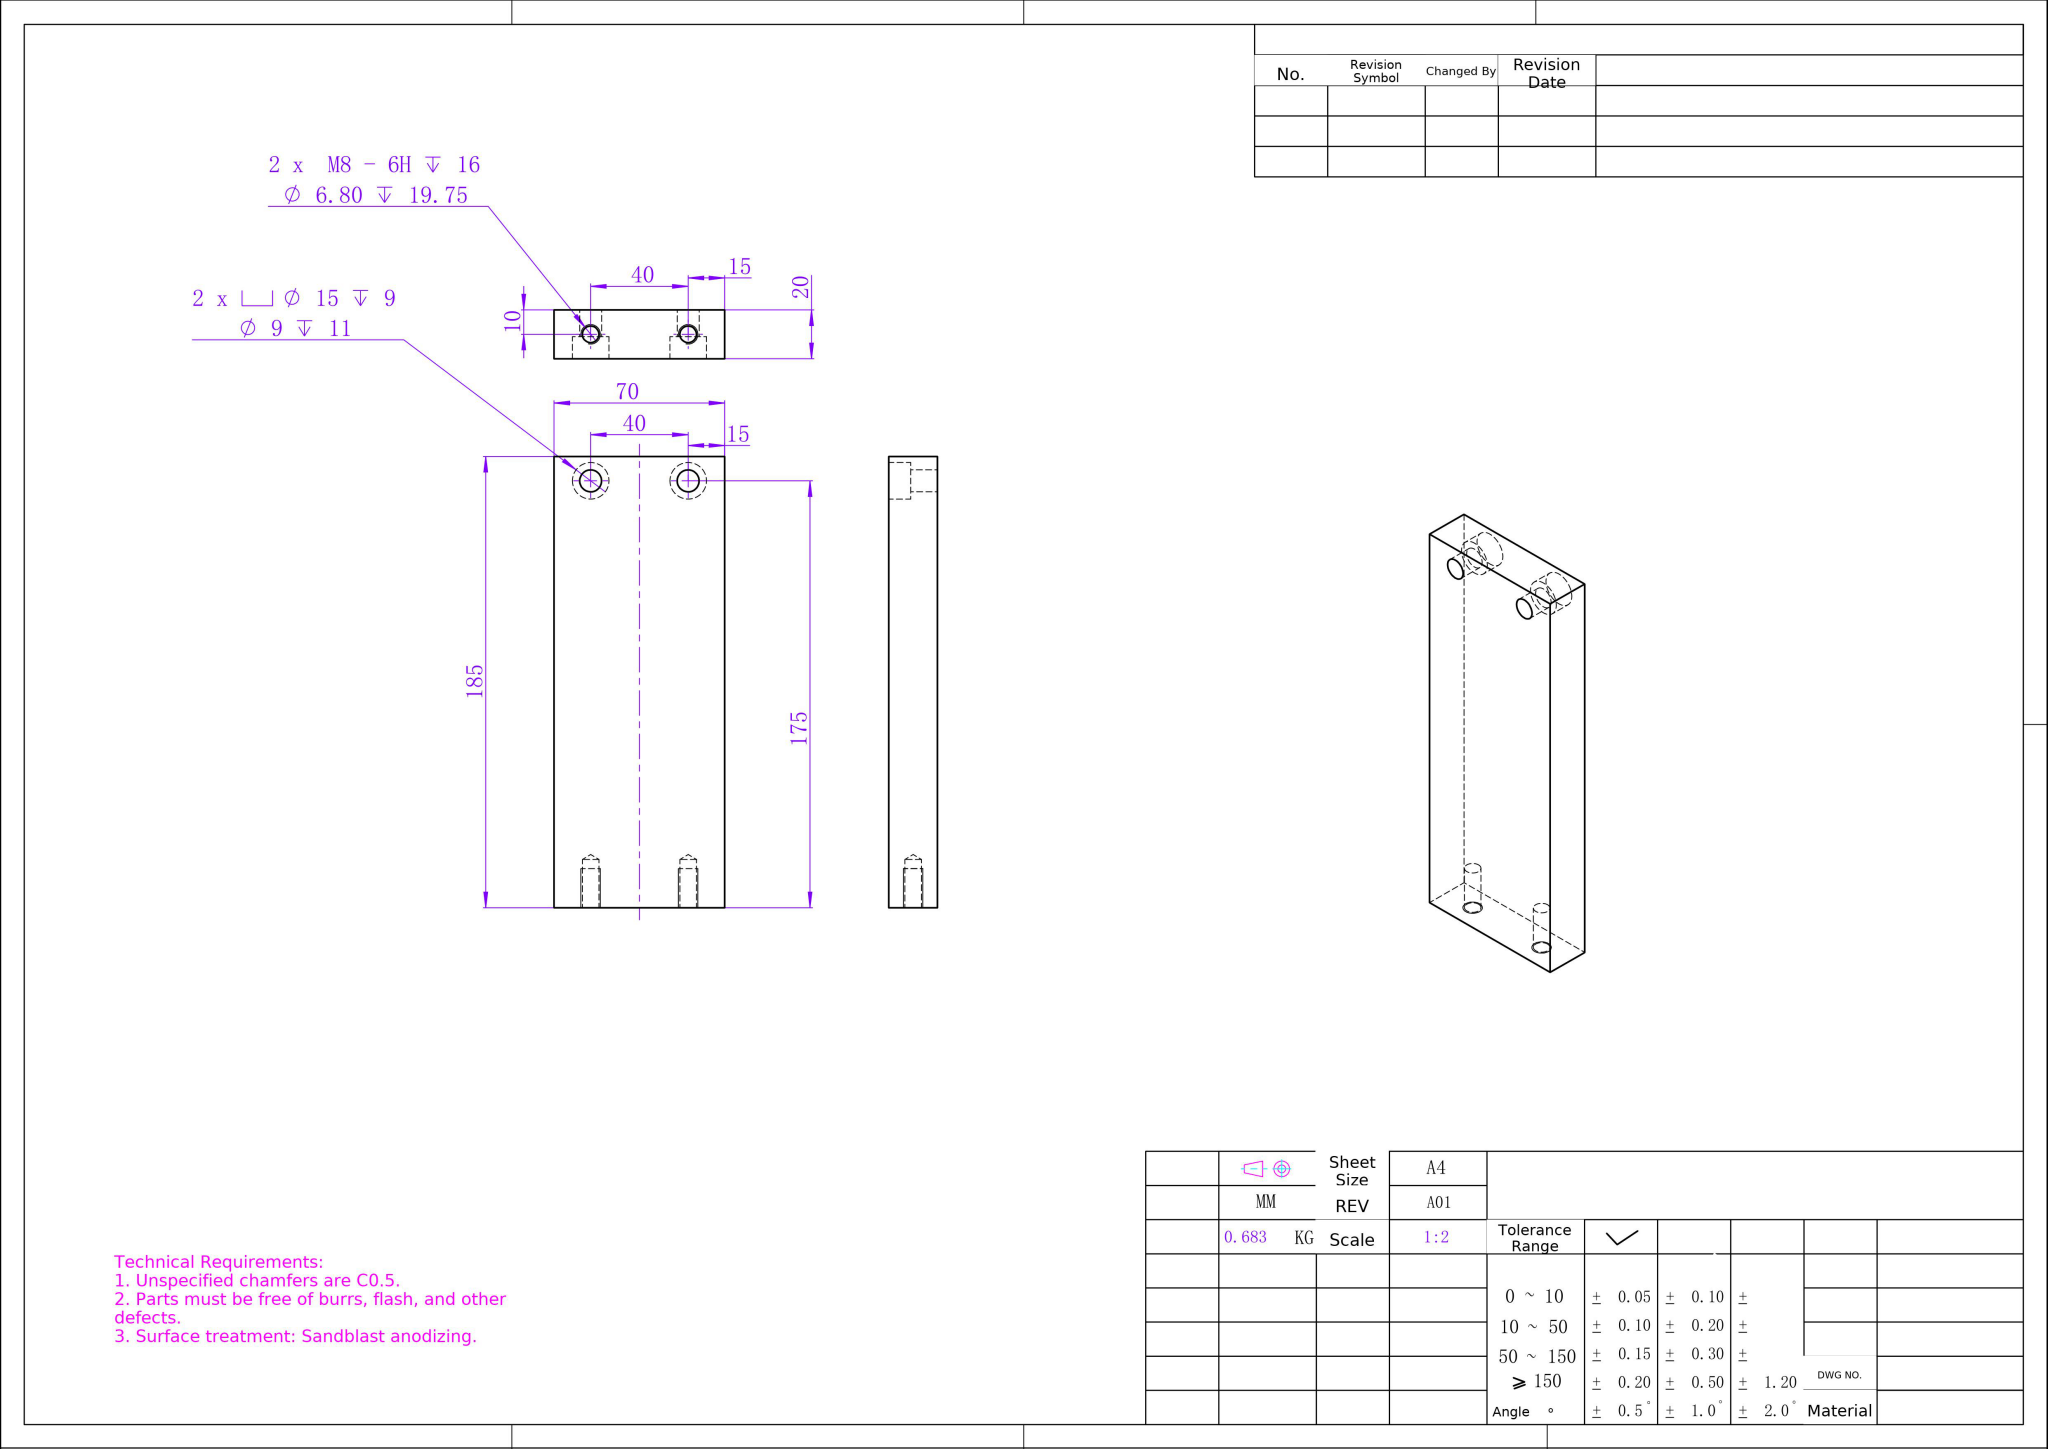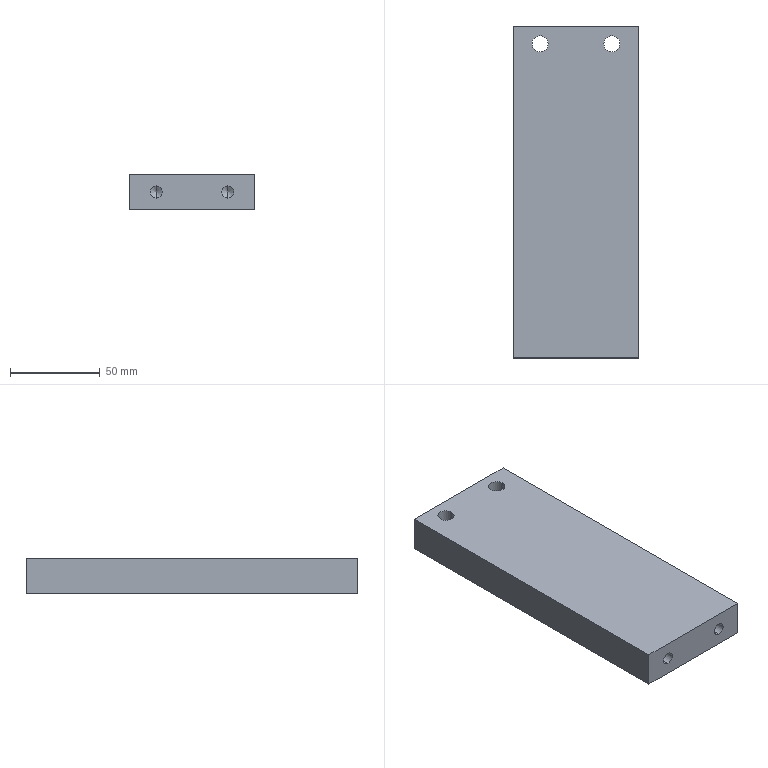Part | NX | mm | 1 solid | 24 faces | box 70 x 185 x 20 mm | volume 252936 mm3 | cylinder 12 | plane 8 | cone 4 | commonest cylinder face diameters 6.8 x4 9 x4 15 x4
STEP:
#1=COLOUR_RGB('',0.0902,1.,0.902);
#2=FILL_AREA_STYLE_COLOUR('',#1);
#3=FILL_AREA_STYLE('',(#2));
#4=SURFACE_STYLE_FILL_AREA(#3);
#5=SURFACE_SIDE_STYLE('',(#4));
#6=SURFACE_STYLE_USAGE(.BOTH.,#5);
#7=PRESENTATION_STYLE_ASSIGNMENT((#6));
#8=CARTESIAN_POINT('',(-695.,514.75,-6.6));
#9=VERTEX_POINT('',#8);
#10=CARTESIAN_POINT('',(-695.,514.75,-13.4));
#11=VERTEX_POINT('',#10);
#12=CARTESIAN_POINT('',(-695.,514.75,-10.));
#13=DIRECTION('',(0.,-1.,0.));
#14=DIRECTION('',(0.,0.,-1.));
#15=AXIS2_PLACEMENT_3D('',#12,#13,#14);
#16=CIRCLE('',#15,3.4);
#17=EDGE_CURVE('',#9,#11,#16,.T.);
#18=ORIENTED_EDGE('',*,*,#17,.F.);
#19=CARTESIAN_POINT('',(-695.,495.,-6.6));
#20=VERTEX_POINT('',#19);
#21=CARTESIAN_POINT('',(-695.,495.,-6.6));
#22=DIRECTION('',(0.,-1.,0.));
#23=VECTOR('',#22,1000.);
#24=LINE('',#21,#23);
#25=EDGE_CURVE('',#9,#20,#24,.T.);
#26=ORIENTED_EDGE('',*,*,#25,.T.);
#27=CARTESIAN_POINT('',(-695.,495.,-13.4));
#28=VERTEX_POINT('',#27);
#29=CARTESIAN_POINT('',(-695.,495.,-10.));
#30=DIRECTION('',(0.,-1.,0.));
#31=DIRECTION('',(0.,0.,-1.));
#32=AXIS2_PLACEMENT_3D('',#29,#30,#31);
#33=CIRCLE('',#32,3.4);
#34=EDGE_CURVE('',#20,#28,#33,.T.);
#35=ORIENTED_EDGE('',*,*,#34,.T.);
#36=CARTESIAN_POINT('',(-695.,495.,-13.4));
#37=DIRECTION('',(0.,-1.,0.));
#38=VECTOR('',#37,1000.);
#39=LINE('',#36,#38);
#40=EDGE_CURVE('',#11,#28,#39,.T.);
#41=ORIENTED_EDGE('',*,*,#40,.F.);
#42=EDGE_LOOP('',(#18,#26,#35,#41));
#43=FACE_OUTER_BOUND('',#42,.T.);
#44=CARTESIAN_POINT('',(-695.,495.,-10.));
#45=DIRECTION('',(0.,-1.,0.));
#46=DIRECTION('',(0.,0.,-1.));
#47=AXIS2_PLACEMENT_3D('',#44,#45,#46);
#48=CYLINDRICAL_SURFACE('',#47,3.4);
#49=ADVANCED_FACE('',(#43),#48,.F.);
#50=STYLED_ITEM('',(#7),#49);
#51=PRESENTATION_LAYER_ASSIGNMENT('','',(#50));
#52=COLOUR_RGB('',0.0902,1.,0.902);
#53=FILL_AREA_STYLE_COLOUR('',#52);
#54=FILL_AREA_STYLE('',(#53));
#55=SURFACE_STYLE_FILL_AREA(#54);
#56=SURFACE_SIDE_STYLE('',(#55));
#57=SURFACE_STYLE_USAGE(.BOTH.,#56);
#58=PRESENTATION_STYLE_ASSIGNMENT((#57));
#59=ORIENTED_EDGE('',*,*,#25,.F.);
#60=CARTESIAN_POINT('',(-695.,514.75,-10.));
#61=DIRECTION('',(0.,-1.,0.));
#62=DIRECTION('',(0.,0.,-1.));
#63=AXIS2_PLACEMENT_3D('',#60,#61,#62);
#64=CIRCLE('',#63,3.4);
#65=EDGE_CURVE('',#11,#9,#64,.T.);
#66=ORIENTED_EDGE('',*,*,#65,.F.);
#67=ORIENTED_EDGE('',*,*,#40,.T.);
#68=CARTESIAN_POINT('',(-695.,495.,-10.));
#69=DIRECTION('',(0.,-1.,0.));
#70=DIRECTION('',(0.,0.,-1.));
#71=AXIS2_PLACEMENT_3D('',#68,#69,#70);
#72=CIRCLE('',#71,3.4);
#73=EDGE_CURVE('',#28,#20,#72,.T.);
#74=ORIENTED_EDGE('',*,*,#73,.T.);
#75=EDGE_LOOP('',(#59,#66,#67,#74));
#76=FACE_OUTER_BOUND('',#75,.T.);
#77=CARTESIAN_POINT('',(-695.,495.,-10.));
#78=DIRECTION('',(0.,-1.,0.));
#79=DIRECTION('',(0.,0.,-1.));
#80=AXIS2_PLACEMENT_3D('',#77,#78,#79);
#81=CYLINDRICAL_SURFACE('',#80,3.4);
#82=ADVANCED_FACE('',(#76),#81,.F.);
#83=STYLED_ITEM('',(#58),#82);
#84=(LENGTH_UNIT()NAMED_UNIT(*)SI_UNIT(.MILLI.,.METRE.));
#85=UNCERTAINTY_MEASURE_WITH_UNIT(LENGTH_MEASURE(0.00001),#84,'','');
#86=(NAMED_UNIT(*)PLANE_ANGLE_UNIT()SI_UNIT($,.RADIAN.));
#87=(NAMED_UNIT(*)SI_UNIT($,.STERADIAN.)SOLID_ANGLE_UNIT());
#88=(GEOMETRIC_REPRESENTATION_CONTEXT(3)GLOBAL_UNCERTAINTY_ASSIGNED_CONTEXT((#85))GLOBAL_UNIT_ASSIGNED_CONTEXT((#84,#86,#87))REPRESENTATION_CONTEXT('',''));
#89=MECHANICAL_DESIGN_GEOMETRIC_PRESENTATION_REPRESENTATION('',(#83),#88);
#90=COLOUR_RGB('',0.0902,1.,0.902);
#91=FILL_AREA_STYLE_COLOUR('',#90);
#92=FILL_AREA_STYLE('',(#91));
#93=SURFACE_STYLE_FILL_AREA(#92);
#94=SURFACE_SIDE_STYLE('',(#93));
#95=SURFACE_STYLE_USAGE(.BOTH.,#94);
#96=PRESENTATION_STYLE_ASSIGNMENT((#95));
#97=CARTESIAN_POINT('',(-695.,516.793,-10.));
#98=VERTEX_POINT('',#97);
#99=CARTESIAN_POINT('',(-695.,514.75,-13.4));
#100=DIRECTION('',(0.,-0.515,-0.8572));
#101=VECTOR('',#100,1000.);
#102=LINE('',#99,#101);
#103=EDGE_CURVE('',#98,#11,#102,.T.);
#104=ORIENTED_EDGE('',*,*,#103,.F.);
#105=CARTESIAN_POINT('',(-695.,514.75,-6.6));
#106=DIRECTION('',(0.,-0.515,0.8572));
#107=VECTOR('',#106,1000.);
#108=LINE('',#105,#107);
#109=EDGE_CURVE('',#98,#9,#108,.T.);
#110=ORIENTED_EDGE('',*,*,#109,.T.);
#111=ORIENTED_EDGE('',*,*,#17,.T.);
#112=EDGE_LOOP('',(#104,#110,#111));
#113=FACE_OUTER_BOUND('',#112,.T.);
#114=CARTESIAN_POINT('',(-695.,514.75,-10.));
#115=DIRECTION('',(0.,-1.,0.));
#116=DIRECTION('',(0.,0.,-1.));
#117=AXIS2_PLACEMENT_3D('',#114,#115,#116);
#118=CONICAL_SURFACE('',#117,3.4,1.03);
#119=ADVANCED_FACE('',(#113),#118,.F.);
#120=CARTESIAN_POINT('',(-735.,514.75,-6.6));
#121=VERTEX_POINT('',#120);
#122=CARTESIAN_POINT('',(-735.,514.75,-13.4));
#123=VERTEX_POINT('',#122);
#124=CARTESIAN_POINT('',(-735.,514.75,-10.));
#125=DIRECTION('',(0.,-1.,0.));
#126=DIRECTION('',(0.,0.,-1.));
#127=AXIS2_PLACEMENT_3D('',#124,#125,#126);
#128=CIRCLE('',#127,3.4);
#129=EDGE_CURVE('',#121,#123,#128,.T.);
#130=ORIENTED_EDGE('',*,*,#129,.F.);
#131=CARTESIAN_POINT('',(-735.,495.,-6.6));
#132=VERTEX_POINT('',#131);
#133=CARTESIAN_POINT('',(-735.,495.,-6.6));
#134=DIRECTION('',(0.,-1.,0.));
#135=VECTOR('',#134,1000.);
#136=LINE('',#133,#135);
#137=EDGE_CURVE('',#121,#132,#136,.T.);
#138=ORIENTED_EDGE('',*,*,#137,.T.);
#139=CARTESIAN_POINT('',(-735.,495.,-13.4));
#140=VERTEX_POINT('',#139);
#141=CARTESIAN_POINT('',(-735.,495.,-10.));
#142=DIRECTION('',(0.,-1.,0.));
#143=DIRECTION('',(0.,0.,-1.));
#144=AXIS2_PLACEMENT_3D('',#141,#142,#143);
#145=CIRCLE('',#144,3.4);
#146=EDGE_CURVE('',#132,#140,#145,.T.);
#147=ORIENTED_EDGE('',*,*,#146,.T.);
#148=CARTESIAN_POINT('',(-735.,495.,-13.4));
#149=DIRECTION('',(0.,-1.,0.));
#150=VECTOR('',#149,1000.);
#151=LINE('',#148,#150);
#152=EDGE_CURVE('',#123,#140,#151,.T.);
#153=ORIENTED_EDGE('',*,*,#152,.F.);
#154=EDGE_LOOP('',(#130,#138,#147,#153));
#155=FACE_OUTER_BOUND('',#154,.T.);
#156=CARTESIAN_POINT('',(-735.,495.,-10.));
#157=DIRECTION('',(0.,-1.,0.));
#158=DIRECTION('',(0.,0.,-1.));
#159=AXIS2_PLACEMENT_3D('',#156,#157,#158);
#160=CYLINDRICAL_SURFACE('',#159,3.4);
#161=ADVANCED_FACE('',(#155),#160,.F.);
#162=CARTESIAN_POINT('',(-735.,516.793,-10.));
#163=VERTEX_POINT('',#162);
#164=CARTESIAN_POINT('',(-735.,514.75,-13.4));
#165=DIRECTION('',(0.,-0.515,-0.8572));
#166=VECTOR('',#165,1000.);
#167=LINE('',#164,#166);
#168=EDGE_CURVE('',#163,#123,#167,.T.);
#169=ORIENTED_EDGE('',*,*,#168,.F.);
#170=CARTESIAN_POINT('',(-735.,514.75,-6.6));
#171=DIRECTION('',(0.,-0.515,0.8572));
#172=VECTOR('',#171,1000.);
#173=LINE('',#170,#172);
#174=EDGE_CURVE('',#163,#121,#173,.T.);
#175=ORIENTED_EDGE('',*,*,#174,.T.);
#176=ORIENTED_EDGE('',*,*,#129,.T.);
#177=EDGE_LOOP('',(#169,#175,#176));
#178=FACE_OUTER_BOUND('',#177,.T.);
#179=CARTESIAN_POINT('',(-735.,514.75,-10.));
#180=DIRECTION('',(0.,-1.,0.));
#181=DIRECTION('',(0.,0.,-1.));
#182=AXIS2_PLACEMENT_3D('',#179,#180,#181);
#183=CONICAL_SURFACE('',#182,3.4,1.03);
#184=ADVANCED_FACE('',(#178),#183,.F.);
#185=CARTESIAN_POINT('',(-730.5,670.,0.));
#186=VERTEX_POINT('',#185);
#187=CARTESIAN_POINT('',(-739.5,670.,0.));
#188=VERTEX_POINT('',#187);
#189=CARTESIAN_POINT('',(-735.,670.,0.));
#190=DIRECTION('',(0.,0.,-1.));
#191=DIRECTION('',(-1.,0.,0.));
#192=AXIS2_PLACEMENT_3D('',#189,#190,#191);
#193=CIRCLE('',#192,4.5);
#194=EDGE_CURVE('',#186,#188,#193,.T.);
#195=ORIENTED_EDGE('',*,*,#194,.F.);
#196=CARTESIAN_POINT('',(-730.5,670.,-11.));
#197=VERTEX_POINT('',#196);
#198=CARTESIAN_POINT('',(-730.5,670.,-20.));
#199=DIRECTION('',(0.,0.,-1.));
#200=VECTOR('',#199,1000.);
#201=LINE('',#198,#200);
#202=EDGE_CURVE('',#186,#197,#201,.T.);
#203=ORIENTED_EDGE('',*,*,#202,.T.);
#204=CARTESIAN_POINT('',(-739.5,670.,-11.));
#205=VERTEX_POINT('',#204);
#206=CARTESIAN_POINT('',(-735.,670.,-11.));
#207=DIRECTION('',(0.,0.,-1.));
#208=DIRECTION('',(-1.,0.,0.));
#209=AXIS2_PLACEMENT_3D('',#206,#207,#208);
#210=CIRCLE('',#209,4.5);
#211=EDGE_CURVE('',#197,#205,#210,.T.);
#212=ORIENTED_EDGE('',*,*,#211,.T.);
#213=CARTESIAN_POINT('',(-739.5,670.,-20.));
#214=DIRECTION('',(0.,0.,-1.));
#215=VECTOR('',#214,1000.);
#216=LINE('',#213,#215);
#217=EDGE_CURVE('',#188,#205,#216,.T.);
#218=ORIENTED_EDGE('',*,*,#217,.F.);
#219=EDGE_LOOP('',(#195,#203,#212,#218));
#220=FACE_OUTER_BOUND('',#219,.T.);
#221=CARTESIAN_POINT('',(-735.,670.,-20.));
#222=DIRECTION('',(0.,0.,-1.));
#223=DIRECTION('',(-1.,0.,0.));
#224=AXIS2_PLACEMENT_3D('',#221,#222,#223);
#225=CYLINDRICAL_SURFACE('',#224,4.5);
#226=ADVANCED_FACE('',(#220),#225,.F.);
#227=CARTESIAN_POINT('',(-727.5,670.,-11.));
#228=VERTEX_POINT('',#227);
#229=CARTESIAN_POINT('',(-742.5,670.,-11.));
#230=VERTEX_POINT('',#229);
#231=CARTESIAN_POINT('',(-735.,670.,-11.));
#232=DIRECTION('',(0.,0.,-1.));
#233=DIRECTION('',(-1.,0.,0.));
#234=AXIS2_PLACEMENT_3D('',#231,#232,#233);
#235=CIRCLE('',#234,7.5);
#236=EDGE_CURVE('',#228,#230,#235,.T.);
#237=ORIENTED_EDGE('',*,*,#236,.F.);
#238=CARTESIAN_POINT('',(-727.5,670.,-20.));
#239=VERTEX_POINT('',#238);
#240=CARTESIAN_POINT('',(-727.5,670.,-20.));
#241=DIRECTION('',(0.,0.,-1.));
#242=VECTOR('',#241,1000.);
#243=LINE('',#240,#242);
#244=EDGE_CURVE('',#228,#239,#243,.T.);
#245=ORIENTED_EDGE('',*,*,#244,.T.);
#246=CARTESIAN_POINT('',(-742.5,670.,-20.));
#247=VERTEX_POINT('',#246);
#248=CARTESIAN_POINT('',(-735.,670.,-20.));
#249=DIRECTION('',(0.,0.,-1.));
#250=DIRECTION('',(-1.,0.,0.));
#251=AXIS2_PLACEMENT_3D('',#248,#249,#250);
#252=CIRCLE('',#251,7.5);
#253=EDGE_CURVE('',#239,#247,#252,.T.);
#254=ORIENTED_EDGE('',*,*,#253,.T.);
#255=CARTESIAN_POINT('',(-742.5,670.,-20.));
#256=DIRECTION('',(0.,0.,-1.));
#257=VECTOR('',#256,1000.);
#258=LINE('',#255,#257);
#259=EDGE_CURVE('',#230,#247,#258,.T.);
#260=ORIENTED_EDGE('',*,*,#259,.F.);
#261=EDGE_LOOP('',(#237,#245,#254,#260));
#262=FACE_OUTER_BOUND('',#261,.T.);
#263=CARTESIAN_POINT('',(-735.,670.,-20.));
#264=DIRECTION('',(0.,0.,-1.));
#265=DIRECTION('',(-1.,0.,0.));
#266=AXIS2_PLACEMENT_3D('',#263,#264,#265);
#267=CYLINDRICAL_SURFACE('',#266,7.5);
#268=ADVANCED_FACE('',(#262),#267,.F.);
#269=CARTESIAN_POINT('',(-690.5,670.,0.));
#270=VERTEX_POINT('',#269);
#271=CARTESIAN_POINT('',(-699.5,670.,0.));
#272=VERTEX_POINT('',#271);
#273=CARTESIAN_POINT('',(-695.,670.,0.));
#274=DIRECTION('',(0.,0.,-1.));
#275=DIRECTION('',(-1.,0.,0.));
#276=AXIS2_PLACEMENT_3D('',#273,#274,#275);
#277=CIRCLE('',#276,4.5);
#278=EDGE_CURVE('',#270,#272,#277,.T.);
#279=ORIENTED_EDGE('',*,*,#278,.F.);
#280=CARTESIAN_POINT('',(-690.5,670.,-11.));
#281=VERTEX_POINT('',#280);
#282=CARTESIAN_POINT('',(-690.5,670.,-20.));
#283=DIRECTION('',(0.,0.,-1.));
#284=VECTOR('',#283,1000.);
#285=LINE('',#282,#284);
#286=EDGE_CURVE('',#270,#281,#285,.T.);
#287=ORIENTED_EDGE('',*,*,#286,.T.);
#288=CARTESIAN_POINT('',(-699.5,670.,-11.));
#289=VERTEX_POINT('',#288);
#290=CARTESIAN_POINT('',(-695.,670.,-11.));
#291=DIRECTION('',(0.,0.,-1.));
#292=DIRECTION('',(-1.,0.,0.));
#293=AXIS2_PLACEMENT_3D('',#290,#291,#292);
#294=CIRCLE('',#293,4.5);
#295=EDGE_CURVE('',#281,#289,#294,.T.);
#296=ORIENTED_EDGE('',*,*,#295,.T.);
#297=CARTESIAN_POINT('',(-699.5,670.,-20.));
#298=DIRECTION('',(0.,0.,-1.));
#299=VECTOR('',#298,1000.);
#300=LINE('',#297,#299);
#301=EDGE_CURVE('',#272,#289,#300,.T.);
#302=ORIENTED_EDGE('',*,*,#301,.F.);
#303=EDGE_LOOP('',(#279,#287,#296,#302));
#304=FACE_OUTER_BOUND('',#303,.T.);
#305=CARTESIAN_POINT('',(-695.,670.,-20.));
#306=DIRECTION('',(0.,0.,-1.));
#307=DIRECTION('',(-1.,0.,0.));
#308=AXIS2_PLACEMENT_3D('',#305,#306,#307);
#309=CYLINDRICAL_SURFACE('',#308,4.5);
#310=ADVANCED_FACE('',(#304),#309,.F.);
#311=CARTESIAN_POINT('',(-687.5,670.,-11.));
#312=VERTEX_POINT('',#311);
#313=CARTESIAN_POINT('',(-702.5,670.,-11.));
#314=VERTEX_POINT('',#313);
#315=CARTESIAN_POINT('',(-695.,670.,-11.));
#316=DIRECTION('',(0.,0.,-1.));
#317=DIRECTION('',(-1.,0.,0.));
#318=AXIS2_PLACEMENT_3D('',#315,#316,#317);
#319=CIRCLE('',#318,7.5);
#320=EDGE_CURVE('',#312,#314,#319,.T.);
#321=ORIENTED_EDGE('',*,*,#320,.F.);
#322=CARTESIAN_POINT('',(-687.5,670.,-20.));
#323=VERTEX_POINT('',#322);
#324=CARTESIAN_POINT('',(-687.5,670.,-20.));
#325=DIRECTION('',(0.,0.,-1.));
#326=VECTOR('',#325,1000.);
#327=LINE('',#324,#326);
#328=EDGE_CURVE('',#312,#323,#327,.T.);
#329=ORIENTED_EDGE('',*,*,#328,.T.);
#330=CARTESIAN_POINT('',(-702.5,670.,-20.));
#331=VERTEX_POINT('',#330);
#332=CARTESIAN_POINT('',(-695.,670.,-20.));
#333=DIRECTION('',(0.,0.,-1.));
#334=DIRECTION('',(-1.,0.,0.));
#335=AXIS2_PLACEMENT_3D('',#332,#333,#334);
#336=CIRCLE('',#335,7.5);
#337=EDGE_CURVE('',#323,#331,#336,.T.);
#338=ORIENTED_EDGE('',*,*,#337,.T.);
#339=CARTESIAN_POINT('',(-702.5,670.,-20.));
#340=DIRECTION('',(0.,0.,-1.));
#341=VECTOR('',#340,1000.);
#342=LINE('',#339,#341);
#343=EDGE_CURVE('',#314,#331,#342,.T.);
#344=ORIENTED_EDGE('',*,*,#343,.F.);
#345=EDGE_LOOP('',(#321,#329,#338,#344));
#346=FACE_OUTER_BOUND('',#345,.T.);
#347=CARTESIAN_POINT('',(-695.,670.,-20.));
#348=DIRECTION('',(0.,0.,-1.));
#349=DIRECTION('',(-1.,0.,0.));
#350=AXIS2_PLACEMENT_3D('',#347,#348,#349);
#351=CYLINDRICAL_SURFACE('',#350,7.5);
#352=ADVANCED_FACE('',(#346),#351,.F.);
#353=CARTESIAN_POINT('',(-750.,680.,-20.));
#354=VERTEX_POINT('',#353);
#355=CARTESIAN_POINT('',(-750.,495.,-20.));
#356=VERTEX_POINT('',#355);
#357=CARTESIAN_POINT('',(-750.,680.,-20.));
#358=DIRECTION('',(0.,-1.,0.));
#359=VECTOR('',#358,1000.);
#360=LINE('',#357,#359);
#361=EDGE_CURVE('',#354,#356,#360,.T.);
#362=ORIENTED_EDGE('',*,*,#361,.T.);
#363=CARTESIAN_POINT('',(-750.,495.,0.));
#364=VERTEX_POINT('',#363);
#365=CARTESIAN_POINT('',(-750.,495.,0.));
#366=DIRECTION('',(0.,0.,-1.));
#367=VECTOR('',#366,1000.);
#368=LINE('',#365,#367);
#369=EDGE_CURVE('',#364,#356,#368,.T.);
#370=ORIENTED_EDGE('',*,*,#369,.F.);
#371=CARTESIAN_POINT('',(-750.,680.,0.));
#372=VERTEX_POINT('',#371);
#373=CARTESIAN_POINT('',(-750.,680.,0.));
#374=DIRECTION('',(0.,-1.,0.));
#375=VECTOR('',#374,1000.);
#376=LINE('',#373,#375);
#377=EDGE_CURVE('',#372,#364,#376,.T.);
#378=ORIENTED_EDGE('',*,*,#377,.F.);
#379=CARTESIAN_POINT('',(-750.,680.,0.));
#380=DIRECTION('',(0.,0.,-1.));
#381=VECTOR('',#380,1000.);
#382=LINE('',#379,#381);
#383=EDGE_CURVE('',#372,#354,#382,.T.);
#384=ORIENTED_EDGE('',*,*,#383,.T.);
#385=EDGE_LOOP('',(#362,#370,#378,#384));
#386=FACE_OUTER_BOUND('',#385,.T.);
#387=CARTESIAN_POINT('',(-750.,680.,0.));
#388=DIRECTION('',(-1.,0.,0.));
#389=DIRECTION('',(0.,0.,1.));
#390=AXIS2_PLACEMENT_3D('',#387,#388,#389);
#391=PLANE('',#390);
#392=ADVANCED_FACE('',(#386),#391,.T.);
#393=CARTESIAN_POINT('',(-680.,495.,0.));
#394=VERTEX_POINT('',#393);
#395=CARTESIAN_POINT('',(-750.,495.,0.));
#396=DIRECTION('',(-1.,0.,0.));
#397=VECTOR('',#396,1000.);
#398=LINE('',#395,#397);
#399=EDGE_CURVE('',#394,#364,#398,.T.);
#400=ORIENTED_EDGE('',*,*,#399,.F.);
#401=CARTESIAN_POINT('',(-680.,680.,0.));
#402=VERTEX_POINT('',#401);
#403=CARTESIAN_POINT('',(-680.,680.,0.));
#404=DIRECTION('',(0.,-1.,0.));
#405=VECTOR('',#404,1000.);
#406=LINE('',#403,#405);
#407=EDGE_CURVE('',#402,#394,#406,.T.);
#408=ORIENTED_EDGE('',*,*,#407,.F.);
#409=CARTESIAN_POINT('',(-750.,680.,0.));
#410=DIRECTION('',(-1.,0.,0.));
#411=VECTOR('',#410,1000.);
#412=LINE('',#409,#411);
#413=EDGE_CURVE('',#402,#372,#412,.T.);
#414=ORIENTED_EDGE('',*,*,#413,.T.);
#415=ORIENTED_EDGE('',*,*,#377,.T.);
#416=EDGE_LOOP('',(#400,#408,#414,#415));
#417=FACE_OUTER_BOUND('',#416,.T.);
#418=CARTESIAN_POINT('',(-735.,670.,0.));
#419=DIRECTION('',(0.,0.,-1.));
#420=DIRECTION('',(-1.,0.,0.));
#421=AXIS2_PLACEMENT_3D('',#418,#419,#420);
#422=CIRCLE('',#421,4.5);
#423=EDGE_CURVE('',#188,#186,#422,.T.);
#424=ORIENTED_EDGE('',*,*,#423,.T.);
#425=ORIENTED_EDGE('',*,*,#194,.T.);
#426=EDGE_LOOP('',(#424,#425));
#427=FACE_BOUND('',#426,.T.);
#428=CARTESIAN_POINT('',(-695.,670.,0.));
#429=DIRECTION('',(0.,0.,-1.));
#430=DIRECTION('',(-1.,0.,0.));
#431=AXIS2_PLACEMENT_3D('',#428,#429,#430);
#432=CIRCLE('',#431,4.5);
#433=EDGE_CURVE('',#272,#270,#432,.T.);
#434=ORIENTED_EDGE('',*,*,#433,.T.);
#435=ORIENTED_EDGE('',*,*,#278,.T.);
#436=EDGE_LOOP('',(#434,#435));
#437=FACE_BOUND('',#436,.T.);
#438=CARTESIAN_POINT('',(-750.,680.,0.));
#439=DIRECTION('',(0.,0.,1.));
#440=DIRECTION('',(1.,0.,0.));
#441=AXIS2_PLACEMENT_3D('',#438,#439,#440);
#442=PLANE('',#441);
#443=ADVANCED_FACE('',(#417,#427,#437),#442,.T.);
#444=ORIENTED_EDGE('',*,*,#407,.T.);
#445=CARTESIAN_POINT('',(-680.,495.,-20.));
#446=VERTEX_POINT('',#445);
#447=CARTESIAN_POINT('',(-680.,495.,0.));
#448=DIRECTION('',(0.,0.,1.));
#449=VECTOR('',#448,1000.);
#450=LINE('',#447,#449);
#451=EDGE_CURVE('',#446,#394,#450,.T.);
#452=ORIENTED_EDGE('',*,*,#451,.F.);
#453=CARTESIAN_POINT('',(-680.,680.,-20.));
#454=VERTEX_POINT('',#453);
#455=CARTESIAN_POINT('',(-680.,680.,-20.));
#456=DIRECTION('',(0.,-1.,0.));
#457=VECTOR('',#456,1000.);
#458=LINE('',#455,#457);
#459=EDGE_CURVE('',#454,#446,#458,.T.);
#460=ORIENTED_EDGE('',*,*,#459,.F.);
#461=CARTESIAN_POINT('',(-680.,680.,0.));
#462=DIRECTION('',(0.,0.,1.));
#463=VECTOR('',#462,1000.);
#464=LINE('',#461,#463);
#465=EDGE_CURVE('',#454,#402,#464,.T.);
#466=ORIENTED_EDGE('',*,*,#465,.T.);
#467=EDGE_LOOP('',(#444,#452,#460,#466));
#468=FACE_OUTER_BOUND('',#467,.T.);
#469=CARTESIAN_POINT('',(-680.,680.,0.));
#470=DIRECTION('',(1.,0.,0.));
#471=DIRECTION('',(0.,0.,-1.));
#472=AXIS2_PLACEMENT_3D('',#469,#470,#471);
#473=PLANE('',#472);
#474=ADVANCED_FACE('',(#468),#473,.T.);
#475=CARTESIAN_POINT('',(-735.,670.,-20.));
#476=DIRECTION('',(0.,0.,-1.));
#477=DIRECTION('',(-1.,0.,0.));
#478=AXIS2_PLACEMENT_3D('',#475,#476,#477);
#479=CIRCLE('',#478,7.5);
#480=EDGE_CURVE('',#247,#239,#479,.T.);
#481=ORIENTED_EDGE('',*,*,#480,.F.);
#482=ORIENTED_EDGE('',*,*,#253,.F.);
#483=EDGE_LOOP('',(#481,#482));
#484=FACE_BOUND('',#483,.T.);
#485=CARTESIAN_POINT('',(-695.,670.,-20.));
#486=DIRECTION('',(0.,0.,-1.));
#487=DIRECTION('',(-1.,0.,0.));
#488=AXIS2_PLACEMENT_3D('',#485,#486,#487);
#489=CIRCLE('',#488,7.5);
#490=EDGE_CURVE('',#331,#323,#489,.T.);
#491=ORIENTED_EDGE('',*,*,#490,.F.);
#492=ORIENTED_EDGE('',*,*,#337,.F.);
#493=EDGE_LOOP('',(#491,#492));
#494=FACE_BOUND('',#493,.T.);
#495=ORIENTED_EDGE('',*,*,#459,.T.);
#496=CARTESIAN_POINT('',(-750.,495.,-20.));
#497=DIRECTION('',(1.,0.,0.));
#498=VECTOR('',#497,1000.);
#499=LINE('',#496,#498);
#500=EDGE_CURVE('',#356,#446,#499,.T.);
#501=ORIENTED_EDGE('',*,*,#500,.F.);
#502=ORIENTED_EDGE('',*,*,#361,.F.);
#503=CARTESIAN_POINT('',(-750.,680.,-20.));
#504=DIRECTION('',(1.,0.,0.));
#505=VECTOR('',#504,1000.);
#506=LINE('',#503,#505);
#507=EDGE_CURVE('',#354,#454,#506,.T.);
#508=ORIENTED_EDGE('',*,*,#507,.T.);
#509=EDGE_LOOP('',(#495,#501,#502,#508));
#510=FACE_OUTER_BOUND('',#509,.T.);
#511=CARTESIAN_POINT('',(-750.,680.,-20.));
#512=DIRECTION('',(0.,0.,-1.));
#513=DIRECTION('',(-1.,0.,0.));
#514=AXIS2_PLACEMENT_3D('',#511,#512,#513);
#515=PLANE('',#514);
#516=ADVANCED_FACE('',(#484,#494,#510),#515,.T.);
#517=ORIENTED_EDGE('',*,*,#383,.F.);
#518=ORIENTED_EDGE('',*,*,#413,.F.);
#519=ORIENTED_EDGE('',*,*,#465,.F.);
#520=ORIENTED_EDGE('',*,*,#507,.F.);
#521=EDGE_LOOP('',(#517,#518,#519,#520));
#522=FACE_OUTER_BOUND('',#521,.T.);
#523=CARTESIAN_POINT('',(0.,680.,0.));
#524=DIRECTION('',(0.,-1.,0.));
#525=DIRECTION('',(0.,0.,-1.));
#526=AXIS2_PLACEMENT_3D('',#523,#524,#525);
#527=PLANE('',#526);
#528=ADVANCED_FACE('',(#522),#527,.F.);
#529=ORIENTED_EDGE('',*,*,#73,.F.);
#530=ORIENTED_EDGE('',*,*,#34,.F.);
#531=EDGE_LOOP('',(#529,#530));
#532=FACE_BOUND('',#531,.T.);
#533=CARTESIAN_POINT('',(-735.,495.,-10.));
#534=DIRECTION('',(0.,-1.,0.));
#535=DIRECTION('',(0.,0.,-1.));
#536=AXIS2_PLACEMENT_3D('',#533,#534,#535);
#537=CIRCLE('',#536,3.4);
#538=EDGE_CURVE('',#140,#132,#537,.T.);
#539=ORIENTED_EDGE('',*,*,#538,.F.);
#540=ORIENTED_EDGE('',*,*,#146,.F.);
#541=EDGE_LOOP('',(#539,#540));
#542=FACE_BOUND('',#541,.T.);
#543=ORIENTED_EDGE('',*,*,#369,.T.);
#544=ORIENTED_EDGE('',*,*,#500,.T.);
#545=ORIENTED_EDGE('',*,*,#451,.T.);
#546=ORIENTED_EDGE('',*,*,#399,.T.);
#547=EDGE_LOOP('',(#543,#544,#545,#546));
#548=FACE_OUTER_BOUND('',#547,.T.);
#549=CARTESIAN_POINT('',(0.,495.,0.));
#550=DIRECTION('',(0.,-1.,0.));
#551=DIRECTION('',(0.,0.,-1.));
#552=AXIS2_PLACEMENT_3D('',#549,#550,#551);
#553=PLANE('',#552);
#554=ADVANCED_FACE('',(#532,#542,#548),#553,.T.);
#555=ORIENTED_EDGE('',*,*,#328,.F.);
#556=CARTESIAN_POINT('',(-695.,670.,-11.));
#557=DIRECTION('',(0.,0.,-1.));
#558=DIRECTION('',(-1.,0.,0.));
#559=AXIS2_PLACEMENT_3D('',#556,#557,#558);
#560=CIRCLE('',#559,7.5);
#561=EDGE_CURVE('',#314,#312,#560,.T.);
#562=ORIENTED_EDGE('',*,*,#561,.F.);
#563=ORIENTED_EDGE('',*,*,#343,.T.);
#564=ORIENTED_EDGE('',*,*,#490,.T.);
#565=EDGE_LOOP('',(#555,#562,#563,#564));
#566=FACE_OUTER_BOUND('',#565,.T.);
#567=CARTESIAN_POINT('',(-695.,670.,-20.));
#568=DIRECTION('',(0.,0.,-1.));
#569=DIRECTION('',(-1.,0.,0.));
#570=AXIS2_PLACEMENT_3D('',#567,#568,#569);
#571=CYLINDRICAL_SURFACE('',#570,7.5);
#572=ADVANCED_FACE('',(#566),#571,.F.);
#573=CARTESIAN_POINT('',(-695.,670.,-11.));
#574=DIRECTION('',(0.,0.,-1.));
#575=DIRECTION('',(-1.,0.,0.));
#576=AXIS2_PLACEMENT_3D('',#573,#574,#575);
#577=CIRCLE('',#576,4.5);
#578=EDGE_CURVE('',#289,#281,#577,.T.);
#579=ORIENTED_EDGE('',*,*,#578,.F.);
#580=ORIENTED_EDGE('',*,*,#295,.F.);
#581=EDGE_LOOP('',(#579,#580));
#582=FACE_BOUND('',#581,.T.);
#583=ORIENTED_EDGE('',*,*,#561,.T.);
#584=ORIENTED_EDGE('',*,*,#320,.T.);
#585=EDGE_LOOP('',(#583,#584));
#586=FACE_OUTER_BOUND('',#585,.T.);
#587=CARTESIAN_POINT('',(-687.5,670.,-11.));
#588=DIRECTION('',(0.,0.,1.));
#589=DIRECTION('',(1.,0.,0.));
#590=AXIS2_PLACEMENT_3D('',#587,#588,#589);
#591=PLANE('',#590);
#592=ADVANCED_FACE('',(#582,#586),#591,.F.);
#593=ORIENTED_EDGE('',*,*,#286,.F.);
#594=ORIENTED_EDGE('',*,*,#433,.F.);
#595=ORIENTED_EDGE('',*,*,#301,.T.);
#596=ORIENTED_EDGE('',*,*,#578,.T.);
#597=EDGE_LOOP('',(#593,#594,#595,#596));
#598=FACE_OUTER_BOUND('',#597,.T.);
#599=CARTESIAN_POINT('',(-695.,670.,-20.));
#600=DIRECTION('',(0.,0.,-1.));
#601=DIRECTION('',(-1.,0.,0.));
#602=AXIS2_PLACEMENT_3D('',#599,#600,#601);
#603=CYLINDRICAL_SURFACE('',#602,4.5);
#604=ADVANCED_FACE('',(#598),#603,.F.);
#605=ORIENTED_EDGE('',*,*,#244,.F.);
#606=CARTESIAN_POINT('',(-735.,670.,-11.));
#607=DIRECTION('',(0.,0.,-1.));
#608=DIRECTION('',(-1.,0.,0.));
#609=AXIS2_PLACEMENT_3D('',#606,#607,#608);
#610=CIRCLE('',#609,7.5);
#611=EDGE_CURVE('',#230,#228,#610,.T.);
#612=ORIENTED_EDGE('',*,*,#611,.F.);
#613=ORIENTED_EDGE('',*,*,#259,.T.);
#614=ORIENTED_EDGE('',*,*,#480,.T.);
#615=EDGE_LOOP('',(#605,#612,#613,#614));
#616=FACE_OUTER_BOUND('',#615,.T.);
#617=CARTESIAN_POINT('',(-735.,670.,-20.));
#618=DIRECTION('',(0.,0.,-1.));
#619=DIRECTION('',(-1.,0.,0.));
#620=AXIS2_PLACEMENT_3D('',#617,#618,#619);
#621=CYLINDRICAL_SURFACE('',#620,7.5);
#622=ADVANCED_FACE('',(#616),#621,.F.);
#623=CARTESIAN_POINT('',(-735.,670.,-11.));
#624=DIRECTION('',(0.,0.,-1.));
#625=DIRECTION('',(-1.,0.,0.));
#626=AXIS2_PLACEMENT_3D('',#623,#624,#625);
#627=CIRCLE('',#626,4.5);
#628=EDGE_CURVE('',#205,#197,#627,.T.);
#629=ORIENTED_EDGE('',*,*,#628,.F.);
#630=ORIENTED_EDGE('',*,*,#211,.F.);
#631=EDGE_LOOP('',(#629,#630));
#632=FACE_BOUND('',#631,.T.);
#633=ORIENTED_EDGE('',*,*,#611,.T.);
#634=ORIENTED_EDGE('',*,*,#236,.T.);
#635=EDGE_LOOP('',(#633,#634));
#636=FACE_OUTER_BOUND('',#635,.T.);
#637=CARTESIAN_POINT('',(-727.5,670.,-11.));
#638=DIRECTION('',(0.,0.,1.));
#639=DIRECTION('',(1.,0.,0.));
#640=AXIS2_PLACEMENT_3D('',#637,#638,#639);
#641=PLANE('',#640);
#642=ADVANCED_FACE('',(#632,#636),#641,.F.);
#643=ORIENTED_EDGE('',*,*,#202,.F.);
#644=ORIENTED_EDGE('',*,*,#423,.F.);
#645=ORIENTED_EDGE('',*,*,#217,.T.);
#646=ORIENTED_EDGE('',*,*,#628,.T.);
#647=EDGE_LOOP('',(#643,#644,#645,#646));
#648=FACE_OUTER_BOUND('',#647,.T.);
#649=CARTESIAN_POINT('',(-735.,670.,-20.));
#650=DIRECTION('',(0.,0.,-1.));
#651=DIRECTION('',(-1.,0.,0.));
#652=AXIS2_PLACEMENT_3D('',#649,#650,#651);
#653=CYLINDRICAL_SURFACE('',#652,4.5);
#654=ADVANCED_FACE('',(#648),#653,.F.);
#655=ORIENTED_EDGE('',*,*,#174,.F.);
#656=ORIENTED_EDGE('',*,*,#168,.T.);
#657=CARTESIAN_POINT('',(-735.,514.75,-10.));
#658=DIRECTION('',(0.,-1.,0.));
#659=DIRECTION('',(0.,0.,-1.));
#660=AXIS2_PLACEMENT_3D('',#657,#658,#659);
#661=CIRCLE('',#660,3.4);
#662=EDGE_CURVE('',#123,#121,#661,.T.);
#663=ORIENTED_EDGE('',*,*,#662,.T.);
#664=EDGE_LOOP('',(#655,#656,#663));
#665=FACE_OUTER_BOUND('',#664,.T.);
#666=CARTESIAN_POINT('',(-735.,514.75,-10.));
#667=DIRECTION('',(0.,-1.,0.));
#668=DIRECTION('',(0.,0.,-1.));
#669=AXIS2_PLACEMENT_3D('',#666,#667,#668);
#670=CONICAL_SURFACE('',#669,3.4,1.03);
#671=ADVANCED_FACE('',(#665),#670,.F.);
#672=ORIENTED_EDGE('',*,*,#137,.F.);
#673=ORIENTED_EDGE('',*,*,#662,.F.);
#674=ORIENTED_EDGE('',*,*,#152,.T.);
#675=ORIENTED_EDGE('',*,*,#538,.T.);
#676=EDGE_LOOP('',(#672,#673,#674,#675));
#677=FACE_OUTER_BOUND('',#676,.T.);
#678=CARTESIAN_POINT('',(-735.,495.,-10.));
#679=DIRECTION('',(0.,-1.,0.));
#680=DIRECTION('',(0.,0.,-1.));
#681=AXIS2_PLACEMENT_3D('',#678,#679,#680);
#682=CYLINDRICAL_SURFACE('',#681,3.4);
#683=ADVANCED_FACE('',(#677),#682,.F.);
#684=ORIENTED_EDGE('',*,*,#109,.F.);
#685=ORIENTED_EDGE('',*,*,#103,.T.);
#686=ORIENTED_EDGE('',*,*,#65,.T.);
#687=EDGE_LOOP('',(#684,#685,#686));
#688=FACE_OUTER_BOUND('',#687,.T.);
#689=CARTESIAN_POINT('',(-695.,514.75,-10.));
#690=DIRECTION('',(0.,-1.,0.));
#691=DIRECTION('',(0.,0.,-1.));
#692=AXIS2_PLACEMENT_3D('',#689,#690,#691);
#693=CONICAL_SURFACE('',#692,3.4,1.03);
#694=ADVANCED_FACE('',(#688),#693,.F.);
#695=CLOSED_SHELL('',(#49,#119,#161,#184,#226,#268,#310,#352,#392,#443,#474,#516,#528,#554,#572,#592,#604,#622,#642,#654,#671,#683,#694,#82));
#696=MANIFOLD_SOLID_BREP('',#695);
#697=CARTESIAN_POINT('',(0.,0.,0.));
#698=DIRECTION('',(0.,0.,1.));
#699=DIRECTION('',(1.,0.,0.));
#700=AXIS2_PLACEMENT_3D('',#697,#698,#699);
#701=(LENGTH_UNIT()NAMED_UNIT(*)SI_UNIT(.MILLI.,.METRE.));
#702=UNCERTAINTY_MEASURE_WITH_UNIT(LENGTH_MEASURE(0.00001),#701,'','');
#703=(NAMED_UNIT(*)PLANE_ANGLE_UNIT()SI_UNIT($,.RADIAN.));
#704=(NAMED_UNIT(*)SI_UNIT($,.STERADIAN.)SOLID_ANGLE_UNIT());
#705=(GEOMETRIC_REPRESENTATION_CONTEXT(3)GLOBAL_UNCERTAINTY_ASSIGNED_CONTEXT((#702))GLOBAL_UNIT_ASSIGNED_CONTEXT((#701,#703,#704))REPRESENTATION_CONTEXT('',''));
#706=ADVANCED_BREP_SHAPE_REPRESENTATION('',(#696,#700),#705);
#707=STYLED_ITEM('',(#96),#706);
#708=PRESENTATION_LAYER_ASSIGNMENT('','',(#707));
#709=(LENGTH_UNIT()NAMED_UNIT(*)SI_UNIT(.MILLI.,.METRE.));
#710=UNCERTAINTY_MEASURE_WITH_UNIT(LENGTH_MEASURE(0.00001),#709,'','');
#711=(NAMED_UNIT(*)PLANE_ANGLE_UNIT()SI_UNIT($,.RADIAN.));
#712=(NAMED_UNIT(*)SI_UNIT($,.STERADIAN.)SOLID_ANGLE_UNIT());
#713=(GEOMETRIC_REPRESENTATION_CONTEXT(3)GLOBAL_UNCERTAINTY_ASSIGNED_CONTEXT((#710))GLOBAL_UNIT_ASSIGNED_CONTEXT((#709,#711,#712))REPRESENTATION_CONTEXT('',''));
#714=MECHANICAL_DESIGN_GEOMETRIC_PRESENTATION_REPRESENTATION('',(#707),#713);
#715=(LENGTH_UNIT()NAMED_UNIT(*)SI_UNIT(.MILLI.,.METRE.));
#716=UNCERTAINTY_MEASURE_WITH_UNIT(LENGTH_MEASURE(0.00001),#715,'','');
#717=(NAMED_UNIT(*)PLANE_ANGLE_UNIT()SI_UNIT($,.RADIAN.));
#718=(NAMED_UNIT(*)SI_UNIT($,.STERADIAN.)SOLID_ANGLE_UNIT());
#719=(GEOMETRIC_REPRESENTATION_CONTEXT(3)GLOBAL_UNCERTAINTY_ASSIGNED_CONTEXT((#716))GLOBAL_UNIT_ASSIGNED_CONTEXT((#715,#717,#718))REPRESENTATION_CONTEXT('',''));
#720=MECHANICAL_DESIGN_GEOMETRIC_PRESENTATION_REPRESENTATION('',(#50),#719);
#721=COLOUR_RGB('',0.0902,1.,0.902);
#722=FILL_AREA_STYLE_COLOUR('',#721);
#723=FILL_AREA_STYLE('',(#722));
#724=SURFACE_STYLE_FILL_AREA(#723);
#725=SURFACE_SIDE_STYLE('',(#724));
#726=SURFACE_STYLE_USAGE(.BOTH.,#725);
#727=PRESENTATION_STYLE_ASSIGNMENT((#726));
#728=STYLED_ITEM('',(#727),#683);
#729=PRESENTATION_LAYER_ASSIGNMENT('','',(#728));
#730=COLOUR_RGB('',0.0902,1.,0.902);
#731=FILL_AREA_STYLE_COLOUR('',#730);
#732=FILL_AREA_STYLE('',(#731));
#733=SURFACE_STYLE_FILL_AREA(#732);
#734=SURFACE_SIDE_STYLE('',(#733));
#735=SURFACE_STYLE_USAGE(.BOTH.,#734);
#736=PRESENTATION_STYLE_ASSIGNMENT((#735));
#737=STYLED_ITEM('',(#736),#161);
#738=(LENGTH_UNIT()NAMED_UNIT(*)SI_UNIT(.MILLI.,.METRE.));
#739=UNCERTAINTY_MEASURE_WITH_UNIT(LENGTH_MEASURE(0.00001),#738,'','');
#740=(NAMED_UNIT(*)PLANE_ANGLE_UNIT()SI_UNIT($,.RADIAN.));
#741=(NAMED_UNIT(*)SI_UNIT($,.STERADIAN.)SOLID_ANGLE_UNIT());
#742=(GEOMETRIC_REPRESENTATION_CONTEXT(3)GLOBAL_UNCERTAINTY_ASSIGNED_CONTEXT((#739))GLOBAL_UNIT_ASSIGNED_CONTEXT((#738,#740,#741))REPRESENTATION_CONTEXT('',''));
#743=MECHANICAL_DESIGN_GEOMETRIC_PRESENTATION_REPRESENTATION('',(#737),#742);
#744=PRESENTATION_LAYER_ASSIGNMENT('','',(#83));
#745=COLOUR_RGB('',0.0902,1.,0.902);
#746=FILL_AREA_STYLE_COLOUR('',#745);
#747=FILL_AREA_STYLE('',(#746));
#748=SURFACE_STYLE_FILL_AREA(#747);
#749=SURFACE_SIDE_STYLE('',(#748));
#750=SURFACE_STYLE_USAGE(.BOTH.,#749);
#751=PRESENTATION_STYLE_ASSIGNMENT((#750));
#752=STYLED_ITEM('',(#751),#696);
#753=PRESENTATION_LAYER_ASSIGNMENT('','',(#752));
#754=(LENGTH_UNIT()NAMED_UNIT(*)SI_UNIT(.MILLI.,.METRE.));
#755=UNCERTAINTY_MEASURE_WITH_UNIT(LENGTH_MEASURE(0.00001),#754,'','');
#756=(NAMED_UNIT(*)PLANE_ANGLE_UNIT()SI_UNIT($,.RADIAN.));
#757=(NAMED_UNIT(*)SI_UNIT($,.STERADIAN.)SOLID_ANGLE_UNIT());
#758=(GEOMETRIC_REPRESENTATION_CONTEXT(3)GLOBAL_UNCERTAINTY_ASSIGNED_CONTEXT((#755))GLOBAL_UNIT_ASSIGNED_CONTEXT((#754,#756,#757))REPRESENTATION_CONTEXT('',''));
#759=MECHANICAL_DESIGN_GEOMETRIC_PRESENTATION_REPRESENTATION('',(#752),#758);
#760=PRESENTATION_LAYER_ASSIGNMENT('','',(#737));
#761=(LENGTH_UNIT()NAMED_UNIT(*)SI_UNIT(.MILLI.,.METRE.));
#762=UNCERTAINTY_MEASURE_WITH_UNIT(LENGTH_MEASURE(0.00001),#761,'','');
#763=(NAMED_UNIT(*)PLANE_ANGLE_UNIT()SI_UNIT($,.RADIAN.));
#764=(NAMED_UNIT(*)SI_UNIT($,.STERADIAN.)SOLID_ANGLE_UNIT());
#765=(GEOMETRIC_REPRESENTATION_CONTEXT(3)GLOBAL_UNCERTAINTY_ASSIGNED_CONTEXT((#762))GLOBAL_UNIT_ASSIGNED_CONTEXT((#761,#763,#764))REPRESENTATION_CONTEXT('',''));
#766=MECHANICAL_DESIGN_GEOMETRIC_PRESENTATION_REPRESENTATION('',(#728),#765);